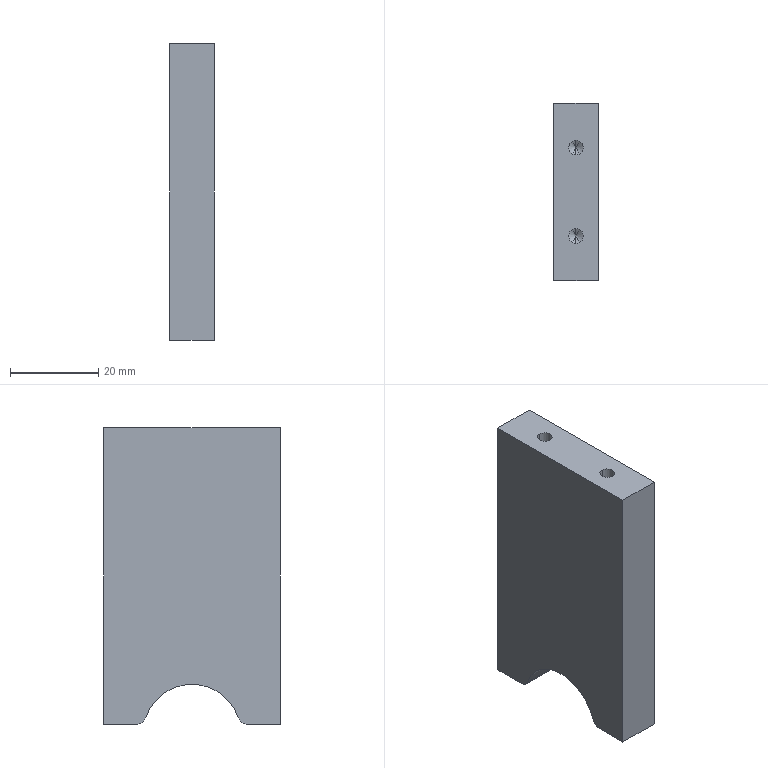Component | SolidWorks | 09-1111-1 | 1 solid | 26 faces | box 10 x 40 x 67 mm | volume 24903 mm3 | cylinder 11 | cone 8 | plane 7 | commonest cylinder face diameters 3.3 x8 4 x2 22 x1 | material AL6061(GB)Natural Anodized
build123d program:
from build123d import *

# Parameters (mm, degrees)
SKETCH1_W             = 67
SKETCH1_H             = 10
EXTRUDE1_DEPTH        = 40
SKETCH2_R             = 11
CUT_EXTRUDE1_DEPTH    = 79.67
M4_TAPPED_HOLE1_D     = 3.3
M4_TAPPED_HOLE1_DEPTH = 12.1
M4_TAPPED_HOLE1_TIP   = 0.9914
M4_TAPPED_HOLE2_D     = 3.3
M4_TAPPED_HOLE2_DEPTH = 12.1
M4_TAPPED_HOLE2_TIP   = 0.9914
FILLET1_R             = 2


with BuildPart() as part:
    # Sketch1 → Extrude1 (new body)
    with BuildSketch(Plane.XY):
        with Locations((33.5, 5)):
            Rectangle(SKETCH1_W, SKETCH1_H)
    extrude(amount=EXTRUDE1_DEPTH)

    # Sketch2 → Cut-Extrude1 (cut, through all)
    with BuildSketch(Plane(origin=(0, 10, 0), x_dir=(1, 0, 0), z_dir=(0, 1, 0))):
        with Locations((-2, -20)):
            Circle(SKETCH2_R)
    extrude(amount=-CUT_EXTRUDE1_DEPTH, mode=Mode.SUBTRACT)

    # M4 Tapped Hole1
    with Locations(Plane(origin=(67, 0, 0), x_dir=(0, 0, -1), z_dir=(1, 0, 0))):
        with Locations((-30, 5), (-10, 5)):
            Hole(M4_TAPPED_HOLE1_D / 2, depth=M4_TAPPED_HOLE1_DEPTH)
            with Locations((0, 0, -(M4_TAPPED_HOLE1_DEPTH + M4_TAPPED_HOLE1_TIP / 2))):  # 118° drill point
                Cone(0, M4_TAPPED_HOLE1_D / 2, M4_TAPPED_HOLE1_TIP, mode=Mode.SUBTRACT)

    # M4 Tapped Hole2
    with Locations(Plane(origin=(0, 5, 3.5), x_dir=(0, 0, -1), z_dir=(-1, 0, 0))):
        with Locations((0, 0), (-33, 0)):
            Hole(M4_TAPPED_HOLE2_D / 2, depth=M4_TAPPED_HOLE2_DEPTH)
            with Locations((0, 0, -(M4_TAPPED_HOLE2_DEPTH + M4_TAPPED_HOLE2_TIP / 2))):  # 118° drill point
                Cone(0, M4_TAPPED_HOLE2_D / 2, M4_TAPPED_HOLE2_TIP, mode=Mode.SUBTRACT)

    # Fillet1
    fillet1_edges = [part.edges().sort_by_distance(p)[0] for p in [
        (0, 5, 9.183),
        (0, 5, 30.817),
    ]]
    fillet(fillet1_edges, radius=FILLET1_R)


solid = part.part

# Placed as in the assembly
solid = solid.moved(Location((105, -35, -73), (90, 0, 90)))
STEP:
#1=CARTESIAN_POINT('',(3.937,-2.88,-2.398));
#2=VERTEX_POINT('',#1);
#3=CARTESIAN_POINT('',(3.937,-2.75,-2.398));
#4=VERTEX_POINT('',#3);
#5=CARTESIAN_POINT('',(3.937,-2.815,-2.398));
#6=DIRECTION('',(0.,-0.,-1.));
#7=DIRECTION('',(0.,1.,0.));
#8=AXIS2_PLACEMENT_3D('',#5,#6,#7);
#9=CIRCLE('',#8,0.06496);
#10=EDGE_CURVE('',#2,#4,#9,.T.);
#11=ORIENTED_EDGE('',*,*,#10,.F.);
#12=CARTESIAN_POINT('',(3.937,-2.88,-2.874));
#13=VERTEX_POINT('',#12);
#14=CARTESIAN_POINT('',(3.937,-2.88,-2.874));
#15=DIRECTION('',(0.,-0.,-1.));
#16=VECTOR('',#15,39.37);
#17=LINE('',#14,#16);
#18=EDGE_CURVE('',#2,#13,#17,.T.);
#19=ORIENTED_EDGE('',*,*,#18,.T.);
#20=CARTESIAN_POINT('',(3.937,-2.75,-2.874));
#21=VERTEX_POINT('',#20);
#22=CARTESIAN_POINT('',(3.937,-2.815,-2.874));
#23=DIRECTION('',(0.,-0.,-1.));
#24=DIRECTION('',(0.,1.,0.));
#25=AXIS2_PLACEMENT_3D('',#22,#23,#24);
#26=CIRCLE('',#25,0.06496);
#27=EDGE_CURVE('',#13,#21,#26,.T.);
#28=ORIENTED_EDGE('',*,*,#27,.T.);
#29=CARTESIAN_POINT('',(3.937,-2.75,-2.874));
#30=DIRECTION('',(0.,-0.,-1.));
#31=VECTOR('',#30,39.37);
#32=LINE('',#29,#31);
#33=EDGE_CURVE('',#4,#21,#32,.T.);
#34=ORIENTED_EDGE('',*,*,#33,.F.);
#35=EDGE_LOOP('',(#11,#19,#28,#34));
#36=FACE_OUTER_BOUND('',#35,.T.);
#37=CARTESIAN_POINT('',(3.937,-2.815,-2.874));
#38=DIRECTION('',(0.,-0.,-1.));
#39=DIRECTION('',(0.,1.,0.));
#40=AXIS2_PLACEMENT_3D('',#37,#38,#39);
#41=CYLINDRICAL_SURFACE('',#40,0.06496);
#42=ADVANCED_FACE('',(#36),#41,.F.);
#43=CARTESIAN_POINT('',(3.937,-2.815,-2.359));
#44=VERTEX_POINT('',#43);
#45=CARTESIAN_POINT('',(3.937,-2.75,-2.398));
#46=DIRECTION('',(0.,0.8572,-0.515));
#47=VECTOR('',#46,39.37);
#48=LINE('',#45,#47);
#49=EDGE_CURVE('',#44,#4,#48,.T.);
#50=ORIENTED_EDGE('',*,*,#49,.F.);
#51=CARTESIAN_POINT('',(3.937,-2.88,-2.398));
#52=DIRECTION('',(0.,-0.8572,-0.515));
#53=VECTOR('',#52,39.37);
#54=LINE('',#51,#53);
#55=EDGE_CURVE('',#44,#2,#54,.T.);
#56=ORIENTED_EDGE('',*,*,#55,.T.);
#57=ORIENTED_EDGE('',*,*,#10,.T.);
#58=EDGE_LOOP('',(#50,#56,#57));
#59=FACE_OUTER_BOUND('',#58,.T.);
#60=CARTESIAN_POINT('',(3.937,-2.815,-2.398));
#61=DIRECTION('',(0.,-0.,-1.));
#62=DIRECTION('',(0.,1.,0.));
#63=AXIS2_PLACEMENT_3D('',#60,#61,#62);
#64=CONICAL_SURFACE('',#63,0.06496,1.03);
#65=ADVANCED_FACE('',(#59),#64,.F.);
#66=CARTESIAN_POINT('',(3.937,-1.581,-2.398));
#67=VERTEX_POINT('',#66);
#68=CARTESIAN_POINT('',(3.937,-1.451,-2.398));
#69=VERTEX_POINT('',#68);
#70=CARTESIAN_POINT('',(3.937,-1.516,-2.398));
#71=DIRECTION('',(0.,-0.,-1.));
#72=DIRECTION('',(0.,1.,0.));
#73=AXIS2_PLACEMENT_3D('',#70,#71,#72);
#74=CIRCLE('',#73,0.06496);
#75=EDGE_CURVE('',#67,#69,#74,.T.);
#76=ORIENTED_EDGE('',*,*,#75,.F.);
#77=CARTESIAN_POINT('',(3.937,-1.581,-2.874));
#78=VERTEX_POINT('',#77);
#79=CARTESIAN_POINT('',(3.937,-1.581,-2.874));
#80=DIRECTION('',(0.,-0.,-1.));
#81=VECTOR('',#80,39.37);
#82=LINE('',#79,#81);
#83=EDGE_CURVE('',#67,#78,#82,.T.);
#84=ORIENTED_EDGE('',*,*,#83,.T.);
#85=CARTESIAN_POINT('',(3.937,-1.451,-2.874));
#86=VERTEX_POINT('',#85);
#87=CARTESIAN_POINT('',(3.937,-1.516,-2.874));
#88=DIRECTION('',(0.,-0.,-1.));
#89=DIRECTION('',(0.,1.,0.));
#90=AXIS2_PLACEMENT_3D('',#87,#88,#89);
#91=CIRCLE('',#90,0.06496);
#92=EDGE_CURVE('',#78,#86,#91,.T.);
#93=ORIENTED_EDGE('',*,*,#92,.T.);
#94=CARTESIAN_POINT('',(3.937,-1.451,-2.874));
#95=DIRECTION('',(0.,-0.,-1.));
#96=VECTOR('',#95,39.37);
#97=LINE('',#94,#96);
#98=EDGE_CURVE('',#69,#86,#97,.T.);
#99=ORIENTED_EDGE('',*,*,#98,.F.);
#100=EDGE_LOOP('',(#76,#84,#93,#99));
#101=FACE_OUTER_BOUND('',#100,.T.);
#102=CARTESIAN_POINT('',(3.937,-1.516,-2.874));
#103=DIRECTION('',(0.,-0.,-1.));
#104=DIRECTION('',(0.,1.,0.));
#105=AXIS2_PLACEMENT_3D('',#102,#103,#104);
#106=CYLINDRICAL_SURFACE('',#105,0.06496);
#107=ADVANCED_FACE('',(#101),#106,.F.);
#108=CARTESIAN_POINT('',(3.937,-1.516,-2.359));
#109=VERTEX_POINT('',#108);
#110=CARTESIAN_POINT('',(3.937,-1.451,-2.398));
#111=DIRECTION('',(0.,0.8572,-0.515));
#112=VECTOR('',#111,39.37);
#113=LINE('',#110,#112);
#114=EDGE_CURVE('',#109,#69,#113,.T.);
#115=ORIENTED_EDGE('',*,*,#114,.F.);
#116=CARTESIAN_POINT('',(3.937,-1.581,-2.398));
#117=DIRECTION('',(0.,-0.8572,-0.515));
#118=VECTOR('',#117,39.37);
#119=LINE('',#116,#118);
#120=EDGE_CURVE('',#109,#67,#119,.T.);
#121=ORIENTED_EDGE('',*,*,#120,.T.);
#122=ORIENTED_EDGE('',*,*,#75,.T.);
#123=EDGE_LOOP('',(#115,#121,#122));
#124=FACE_OUTER_BOUND('',#123,.T.);
#125=CARTESIAN_POINT('',(3.937,-1.516,-2.398));
#126=DIRECTION('',(0.,-0.,-1.));
#127=DIRECTION('',(0.,1.,0.));
#128=AXIS2_PLACEMENT_3D('',#125,#126,#127);
#129=CONICAL_SURFACE('',#128,0.06496,1.03);
#130=ADVANCED_FACE('',(#124),#129,.F.);
#131=CARTESIAN_POINT('',(3.937,-1.707,-0.7126));
#132=VERTEX_POINT('',#131);
#133=CARTESIAN_POINT('',(3.937,-1.837,-0.7126));
#134=VERTEX_POINT('',#133);
#135=CARTESIAN_POINT('',(3.937,-1.772,-0.7126));
#136=DIRECTION('',(-0.,0.,1.));
#137=DIRECTION('',(0.,-1.,0.));
#138=AXIS2_PLACEMENT_3D('',#135,#136,#137);
#139=CIRCLE('',#138,0.06496);
#140=EDGE_CURVE('',#132,#134,#139,.T.);
#141=ORIENTED_EDGE('',*,*,#140,.F.);
#142=CARTESIAN_POINT('',(3.937,-1.707,-0.2362));
#143=VERTEX_POINT('',#142);
#144=CARTESIAN_POINT('',(3.937,-1.707,-0.2362));
#145=DIRECTION('',(-0.,0.,1.));
#146=VECTOR('',#145,39.37);
#147=LINE('',#144,#146);
#148=EDGE_CURVE('',#132,#143,#147,.T.);
#149=ORIENTED_EDGE('',*,*,#148,.T.);
#150=CARTESIAN_POINT('',(3.937,-1.837,-0.2362));
#151=VERTEX_POINT('',#150);
#152=CARTESIAN_POINT('',(3.937,-1.772,-0.2362));
#153=DIRECTION('',(-0.,0.,1.));
#154=DIRECTION('',(0.,-1.,0.));
#155=AXIS2_PLACEMENT_3D('',#152,#153,#154);
#156=CIRCLE('',#155,0.06496);
#157=EDGE_CURVE('',#143,#151,#156,.T.);
#158=ORIENTED_EDGE('',*,*,#157,.T.);
#159=CARTESIAN_POINT('',(3.937,-1.837,-0.2362));
#160=DIRECTION('',(-0.,0.,1.));
#161=VECTOR('',#160,39.37);
#162=LINE('',#159,#161);
#163=EDGE_CURVE('',#134,#151,#162,.T.);
#164=ORIENTED_EDGE('',*,*,#163,.F.);
#165=EDGE_LOOP('',(#141,#149,#158,#164));
#166=FACE_OUTER_BOUND('',#165,.T.);
#167=CARTESIAN_POINT('',(3.937,-1.772,-0.2362));
#168=DIRECTION('',(-0.,0.,1.));
#169=DIRECTION('',(0.,-1.,0.));
#170=AXIS2_PLACEMENT_3D('',#167,#168,#169);
#171=CYLINDRICAL_SURFACE('',#170,0.06496);
#172=ADVANCED_FACE('',(#166),#171,.F.);
#173=CARTESIAN_POINT('',(3.937,-1.772,-0.7516));
#174=VERTEX_POINT('',#173);
#175=CARTESIAN_POINT('',(3.937,-1.837,-0.7126));
#176=DIRECTION('',(-0.,-0.8572,0.515));
#177=VECTOR('',#176,39.37);
#178=LINE('',#175,#177);
#179=EDGE_CURVE('',#174,#134,#178,.T.);
#180=ORIENTED_EDGE('',*,*,#179,.F.);
#181=CARTESIAN_POINT('',(3.937,-1.707,-0.7126));
#182=DIRECTION('',(0.,0.8572,0.515));
#183=VECTOR('',#182,39.37);
#184=LINE('',#181,#183);
#185=EDGE_CURVE('',#174,#132,#184,.T.);
#186=ORIENTED_EDGE('',*,*,#185,.T.);
#187=ORIENTED_EDGE('',*,*,#140,.T.);
#188=EDGE_LOOP('',(#180,#186,#187));
#189=FACE_OUTER_BOUND('',#188,.T.);
#190=CARTESIAN_POINT('',(3.937,-1.772,-0.7126));
#191=DIRECTION('',(-0.,0.,1.));
#192=DIRECTION('',(0.,-1.,0.));
#193=AXIS2_PLACEMENT_3D('',#190,#191,#192);
#194=CONICAL_SURFACE('',#193,0.06496,1.03);
#195=ADVANCED_FACE('',(#189),#194,.F.);
#196=CARTESIAN_POINT('',(3.937,-2.494,-0.7126));
#197=VERTEX_POINT('',#196);
#198=CARTESIAN_POINT('',(3.937,-2.624,-0.7126));
#199=VERTEX_POINT('',#198);
#200=CARTESIAN_POINT('',(3.937,-2.559,-0.7126));
#201=DIRECTION('',(-0.,0.,1.));
#202=DIRECTION('',(0.,-1.,0.));
#203=AXIS2_PLACEMENT_3D('',#200,#201,#202);
#204=CIRCLE('',#203,0.06496);
#205=EDGE_CURVE('',#197,#199,#204,.T.);
#206=ORIENTED_EDGE('',*,*,#205,.F.);
#207=CARTESIAN_POINT('',(3.937,-2.494,-0.2362));
#208=VERTEX_POINT('',#207);
#209=CARTESIAN_POINT('',(3.937,-2.494,-0.2362));
#210=DIRECTION('',(-0.,0.,1.));
#211=VECTOR('',#210,39.37);
#212=LINE('',#209,#211);
#213=EDGE_CURVE('',#197,#208,#212,.T.);
#214=ORIENTED_EDGE('',*,*,#213,.T.);
#215=CARTESIAN_POINT('',(3.937,-2.624,-0.2362));
#216=VERTEX_POINT('',#215);
#217=CARTESIAN_POINT('',(3.937,-2.559,-0.2362));
#218=DIRECTION('',(-0.,0.,1.));
#219=DIRECTION('',(0.,-1.,0.));
#220=AXIS2_PLACEMENT_3D('',#217,#218,#219);
#221=CIRCLE('',#220,0.06496);
#222=EDGE_CURVE('',#208,#216,#221,.T.);
#223=ORIENTED_EDGE('',*,*,#222,.T.);
#224=CARTESIAN_POINT('',(3.937,-2.624,-0.2362));
#225=DIRECTION('',(-0.,0.,1.));
#226=VECTOR('',#225,39.37);
#227=LINE('',#224,#226);
#228=EDGE_CURVE('',#199,#216,#227,.T.);
#229=ORIENTED_EDGE('',*,*,#228,.F.);
#230=EDGE_LOOP('',(#206,#214,#223,#229));
#231=FACE_OUTER_BOUND('',#230,.T.);
#232=CARTESIAN_POINT('',(3.937,-2.559,-0.2362));
#233=DIRECTION('',(-0.,0.,1.));
#234=DIRECTION('',(0.,-1.,0.));
#235=AXIS2_PLACEMENT_3D('',#232,#233,#234);
#236=CYLINDRICAL_SURFACE('',#235,0.06496);
#237=ADVANCED_FACE('',(#231),#236,.F.);
#238=CARTESIAN_POINT('',(3.937,-2.559,-0.7516));
#239=VERTEX_POINT('',#238);
#240=CARTESIAN_POINT('',(3.937,-2.624,-0.7126));
#241=DIRECTION('',(-0.,-0.8572,0.515));
#242=VECTOR('',#241,39.37);
#243=LINE('',#240,#242);
#244=EDGE_CURVE('',#239,#199,#243,.T.);
#245=ORIENTED_EDGE('',*,*,#244,.F.);
#246=CARTESIAN_POINT('',(3.937,-2.494,-0.7126));
#247=DIRECTION('',(0.,0.8572,0.515));
#248=VECTOR('',#247,39.37);
#249=LINE('',#246,#248);
#250=EDGE_CURVE('',#239,#197,#249,.T.);
#251=ORIENTED_EDGE('',*,*,#250,.T.);
#252=ORIENTED_EDGE('',*,*,#205,.T.);
#253=EDGE_LOOP('',(#245,#251,#252));
#254=FACE_OUTER_BOUND('',#253,.T.);
#255=CARTESIAN_POINT('',(3.937,-2.559,-0.7126));
#256=DIRECTION('',(-0.,0.,1.));
#257=DIRECTION('',(0.,-1.,0.));
#258=AXIS2_PLACEMENT_3D('',#255,#256,#257);
#259=CONICAL_SURFACE('',#258,0.06496,1.03);
#260=ADVANCED_FACE('',(#254),#259,.F.);
#261=CARTESIAN_POINT('',(3.937,-2.815,-2.874));
#262=DIRECTION('',(0.,-0.,-1.));
#263=DIRECTION('',(0.,1.,0.));
#264=AXIS2_PLACEMENT_3D('',#261,#262,#263);
#265=CIRCLE('',#264,0.06496);
#266=EDGE_CURVE('',#21,#13,#265,.T.);
#267=ORIENTED_EDGE('',*,*,#266,.F.);
#268=ORIENTED_EDGE('',*,*,#27,.F.);
#269=EDGE_LOOP('',(#267,#268));
#270=FACE_BOUND('',#269,.T.);
#271=CARTESIAN_POINT('',(3.74,-2.652,-2.874));
#272=VERTEX_POINT('',#271);
#273=CARTESIAN_POINT('',(3.74,-2.953,-2.874));
#274=VERTEX_POINT('',#273);
#275=CARTESIAN_POINT('',(3.74,-1.378,-2.874));
#276=DIRECTION('',(-0.,-1.,0.));
#277=VECTOR('',#276,39.37);
#278=LINE('',#275,#277);
#279=EDGE_CURVE('',#272,#274,#278,.T.);
#280=ORIENTED_EDGE('',*,*,#279,.F.);
#281=CARTESIAN_POINT('',(4.134,-2.652,-2.874));
#282=VERTEX_POINT('',#281);
#283=CARTESIAN_POINT('',(3.74,-2.652,-2.874));
#284=DIRECTION('',(1.,-0.,0.));
#285=VECTOR('',#284,39.37);
#286=LINE('',#283,#285);
#287=EDGE_CURVE('',#272,#282,#286,.T.);
#288=ORIENTED_EDGE('',*,*,#287,.T.);
#289=CARTESIAN_POINT('',(4.134,-2.953,-2.874));
#290=VERTEX_POINT('',#289);
#291=CARTESIAN_POINT('',(4.134,-1.378,-2.874));
#292=DIRECTION('',(-0.,-1.,0.));
#293=VECTOR('',#292,39.37);
#294=LINE('',#291,#293);
#295=EDGE_CURVE('',#282,#290,#294,.T.);
#296=ORIENTED_EDGE('',*,*,#295,.T.);
#297=CARTESIAN_POINT('',(3.74,-2.953,-2.874));
#298=DIRECTION('',(-1.,0.,-0.));
#299=VECTOR('',#298,39.37);
#300=LINE('',#297,#299);
#301=EDGE_CURVE('',#290,#274,#300,.T.);
#302=ORIENTED_EDGE('',*,*,#301,.T.);
#303=EDGE_LOOP('',(#280,#288,#296,#302));
#304=FACE_OUTER_BOUND('',#303,.T.);
#305=CARTESIAN_POINT('',(3.74,-1.378,-2.874));
#306=DIRECTION('',(-0.,0.,1.));
#307=DIRECTION('',(-0.,-1.,0.));
#308=AXIS2_PLACEMENT_3D('',#305,#306,#307);
#309=PLANE('',#308);
#310=ADVANCED_FACE('',(#270,#304),#309,.F.);
#311=CARTESIAN_POINT('',(3.937,-1.516,-2.874));
#312=DIRECTION('',(0.,-0.,-1.));
#313=DIRECTION('',(0.,1.,0.));
#314=AXIS2_PLACEMENT_3D('',#311,#312,#313);
#315=CIRCLE('',#314,0.06496);
#316=EDGE_CURVE('',#86,#78,#315,.T.);
#317=ORIENTED_EDGE('',*,*,#316,.F.);
#318=ORIENTED_EDGE('',*,*,#92,.F.);
#319=EDGE_LOOP('',(#317,#318));
#320=FACE_BOUND('',#319,.T.);
#321=CARTESIAN_POINT('',(4.134,-1.378,-2.874));
#322=VERTEX_POINT('',#321);
#323=CARTESIAN_POINT('',(4.134,-1.678,-2.874));
#324=VERTEX_POINT('',#323);
#325=CARTESIAN_POINT('',(4.134,-1.378,-2.874));
#326=DIRECTION('',(-0.,-1.,0.));
#327=VECTOR('',#326,39.37);
#328=LINE('',#325,#327);
#329=EDGE_CURVE('',#322,#324,#328,.T.);
#330=ORIENTED_EDGE('',*,*,#329,.T.);
#331=CARTESIAN_POINT('',(3.74,-1.678,-2.874));
#332=VERTEX_POINT('',#331);
#333=CARTESIAN_POINT('',(3.74,-1.678,-2.874));
#334=DIRECTION('',(-1.,0.,-0.));
#335=VECTOR('',#334,39.37);
#336=LINE('',#333,#335);
#337=EDGE_CURVE('',#324,#332,#336,.T.);
#338=ORIENTED_EDGE('',*,*,#337,.T.);
#339=CARTESIAN_POINT('',(3.74,-1.378,-2.874));
#340=VERTEX_POINT('',#339);
#341=CARTESIAN_POINT('',(3.74,-1.378,-2.874));
#342=DIRECTION('',(-0.,-1.,0.));
#343=VECTOR('',#342,39.37);
#344=LINE('',#341,#343);
#345=EDGE_CURVE('',#340,#332,#344,.T.);
#346=ORIENTED_EDGE('',*,*,#345,.F.);
#347=CARTESIAN_POINT('',(3.74,-1.378,-2.874));
#348=DIRECTION('',(-1.,0.,-0.));
#349=VECTOR('',#348,39.37);
#350=LINE('',#347,#349);
#351=EDGE_CURVE('',#322,#340,#350,.T.);
#352=ORIENTED_EDGE('',*,*,#351,.F.);
#353=EDGE_LOOP('',(#330,#338,#346,#352));
#354=FACE_OUTER_BOUND('',#353,.T.);
#355=CARTESIAN_POINT('',(3.74,-1.378,-2.874));
#356=DIRECTION('',(-0.,0.,1.));
#357=DIRECTION('',(-0.,-1.,0.));
#358=AXIS2_PLACEMENT_3D('',#355,#356,#357);
#359=PLANE('',#358);
#360=ADVANCED_FACE('',(#320,#354),#359,.F.);
#361=ORIENTED_EDGE('',*,*,#345,.T.);
#362=CARTESIAN_POINT('',(3.74,-1.753,-2.82));
#363=VERTEX_POINT('',#362);
#364=CARTESIAN_POINT('',(3.74,-1.678,-2.795));
#365=DIRECTION('',(-1.,0.,-0.));
#366=DIRECTION('',(0.,1.,0.));
#367=AXIS2_PLACEMENT_3D('',#364,#365,#366);
#368=CIRCLE('',#367,0.07874);
#369=EDGE_CURVE('',#332,#363,#368,.T.);
#370=ORIENTED_EDGE('',*,*,#369,.T.);
#371=CARTESIAN_POINT('',(3.74,-2.577,-2.82));
#372=VERTEX_POINT('',#371);
#373=CARTESIAN_POINT('',(3.74,-2.165,-2.953));
#374=DIRECTION('',(1.,-0.,0.));
#375=DIRECTION('',(0.,1.,0.));
#376=AXIS2_PLACEMENT_3D('',#373,#374,#375);
#377=CIRCLE('',#376,0.4331);
#378=EDGE_CURVE('',#363,#372,#377,.T.);
#379=ORIENTED_EDGE('',*,*,#378,.T.);
#380=CARTESIAN_POINT('',(3.74,-2.652,-2.795));
#381=DIRECTION('',(-1.,0.,-0.));
#382=DIRECTION('',(0.,1.,0.));
#383=AXIS2_PLACEMENT_3D('',#380,#381,#382);
#384=CIRCLE('',#383,0.07874);
#385=EDGE_CURVE('',#372,#272,#384,.T.);
#386=ORIENTED_EDGE('',*,*,#385,.T.);
#387=ORIENTED_EDGE('',*,*,#279,.T.);
#388=CARTESIAN_POINT('',(3.74,-2.953,-0.2362));
#389=VERTEX_POINT('',#388);
#390=CARTESIAN_POINT('',(3.74,-2.953,-2.874));
#391=DIRECTION('',(-0.,0.,1.));
#392=VECTOR('',#391,39.37);
#393=LINE('',#390,#392);
#394=EDGE_CURVE('',#274,#389,#393,.T.);
#395=ORIENTED_EDGE('',*,*,#394,.T.);
#396=CARTESIAN_POINT('',(3.74,-1.378,-0.2362));
#397=VERTEX_POINT('',#396);
#398=CARTESIAN_POINT('',(3.74,-1.378,-0.2362));
#399=DIRECTION('',(-0.,-1.,0.));
#400=VECTOR('',#399,39.37);
#401=LINE('',#398,#400);
#402=EDGE_CURVE('',#397,#389,#401,.T.);
#403=ORIENTED_EDGE('',*,*,#402,.F.);
#404=CARTESIAN_POINT('',(3.74,-1.378,-2.874));
#405=DIRECTION('',(-0.,0.,1.));
#406=VECTOR('',#405,39.37);
#407=LINE('',#404,#406);
#408=EDGE_CURVE('',#340,#397,#407,.T.);
#409=ORIENTED_EDGE('',*,*,#408,.F.);
#410=EDGE_LOOP('',(#361,#370,#379,#386,#387,#395,#403,#409));
#411=FACE_OUTER_BOUND('',#410,.T.);
#412=CARTESIAN_POINT('',(3.74,-1.378,-2.874));
#413=DIRECTION('',(1.,-0.,0.));
#414=DIRECTION('',(0.,1.,-0.));
#415=AXIS2_PLACEMENT_3D('',#412,#413,#414);
#416=PLANE('',#415);
#417=ADVANCED_FACE('',(#411),#416,.F.);
#418=CARTESIAN_POINT('',(3.937,-1.772,-0.2362));
#419=DIRECTION('',(-0.,0.,1.));
#420=DIRECTION('',(0.,-1.,0.));
#421=AXIS2_PLACEMENT_3D('',#418,#419,#420);
#422=CIRCLE('',#421,0.06496);
#423=EDGE_CURVE('',#151,#143,#422,.T.);
#424=ORIENTED_EDGE('',*,*,#423,.F.);
#425=ORIENTED_EDGE('',*,*,#157,.F.);
#426=EDGE_LOOP('',(#424,#425));
#427=FACE_BOUND('',#426,.T.);
#428=CARTESIAN_POINT('',(3.937,-2.559,-0.2362));
#429=DIRECTION('',(-0.,0.,1.));
#430=DIRECTION('',(0.,-1.,0.));
#431=AXIS2_PLACEMENT_3D('',#428,#429,#430);
#432=CIRCLE('',#431,0.06496);
#433=EDGE_CURVE('',#216,#208,#432,.T.);
#434=ORIENTED_EDGE('',*,*,#433,.F.);
#435=ORIENTED_EDGE('',*,*,#222,.F.);
#436=EDGE_LOOP('',(#434,#435));
#437=FACE_BOUND('',#436,.T.);
#438=CARTESIAN_POINT('',(4.134,-2.953,-0.2362));
#439=VERTEX_POINT('',#438);
#440=CARTESIAN_POINT('',(3.74,-2.953,-0.2362));
#441=DIRECTION('',(1.,-0.,0.));
#442=VECTOR('',#441,39.37);
#443=LINE('',#440,#442);
#444=EDGE_CURVE('',#389,#439,#443,.T.);
#445=ORIENTED_EDGE('',*,*,#444,.T.);
#446=CARTESIAN_POINT('',(4.134,-1.378,-0.2362));
#447=VERTEX_POINT('',#446);
#448=CARTESIAN_POINT('',(4.134,-1.378,-0.2362));
#449=DIRECTION('',(-0.,-1.,0.));
#450=VECTOR('',#449,39.37);
#451=LINE('',#448,#450);
#452=EDGE_CURVE('',#447,#439,#451,.T.);
#453=ORIENTED_EDGE('',*,*,#452,.F.);
#454=CARTESIAN_POINT('',(3.74,-1.378,-0.2362));
#455=DIRECTION('',(1.,-0.,0.));
#456=VECTOR('',#455,39.37);
#457=LINE('',#454,#456);
#458=EDGE_CURVE('',#397,#447,#457,.T.);
#459=ORIENTED_EDGE('',*,*,#458,.F.);
#460=ORIENTED_EDGE('',*,*,#402,.T.);
#461=EDGE_LOOP('',(#445,#453,#459,#460));
#462=FACE_OUTER_BOUND('',#461,.T.);
#463=CARTESIAN_POINT('',(3.74,-1.378,-0.2362));
#464=DIRECTION('',(0.,-0.,-1.));
#465=DIRECTION('',(0.,1.,-0.));
#466=AXIS2_PLACEMENT_3D('',#463,#464,#465);
#467=PLANE('',#466);
#468=ADVANCED_FACE('',(#427,#437,#462),#467,.F.);
#469=CARTESIAN_POINT('',(4.134,-1.753,-2.82));
#470=VERTEX_POINT('',#469);
#471=CARTESIAN_POINT('',(4.134,-2.577,-2.82));
#472=VERTEX_POINT('',#471);
#473=CARTESIAN_POINT('',(4.134,-2.165,-2.953));
#474=DIRECTION('',(1.,-0.,0.));
#475=DIRECTION('',(0.,1.,0.));
#476=AXIS2_PLACEMENT_3D('',#473,#474,#475);
#477=CIRCLE('',#476,0.4331);
#478=EDGE_CURVE('',#470,#472,#477,.T.);
#479=ORIENTED_EDGE('',*,*,#478,.F.);
#480=CARTESIAN_POINT('',(4.134,-1.678,-2.795));
#481=DIRECTION('',(1.,-0.,0.));
#482=DIRECTION('',(0.,-1.,0.));
#483=AXIS2_PLACEMENT_3D('',#480,#481,#482);
#484=CIRCLE('',#483,0.07874);
#485=EDGE_CURVE('',#470,#324,#484,.T.);
#486=ORIENTED_EDGE('',*,*,#485,.T.);
#487=ORIENTED_EDGE('',*,*,#329,.F.);
#488=CARTESIAN_POINT('',(4.134,-1.378,-2.874));
#489=DIRECTION('',(0.,-0.,-1.));
#490=VECTOR('',#489,39.37);
#491=LINE('',#488,#490);
#492=EDGE_CURVE('',#447,#322,#491,.T.);
#493=ORIENTED_EDGE('',*,*,#492,.F.);
#494=ORIENTED_EDGE('',*,*,#452,.T.);
#495=CARTESIAN_POINT('',(4.134,-2.953,-2.874));
#496=DIRECTION('',(0.,-0.,-1.));
#497=VECTOR('',#496,39.37);
#498=LINE('',#495,#497);
#499=EDGE_CURVE('',#439,#290,#498,.T.);
#500=ORIENTED_EDGE('',*,*,#499,.T.);
#501=ORIENTED_EDGE('',*,*,#295,.F.);
#502=CARTESIAN_POINT('',(4.134,-2.652,-2.795));
#503=DIRECTION('',(1.,-0.,0.));
#504=DIRECTION('',(0.,-1.,0.));
#505=AXIS2_PLACEMENT_3D('',#502,#503,#504);
#506=CIRCLE('',#505,0.07874);
#507=EDGE_CURVE('',#282,#472,#506,.T.);
#508=ORIENTED_EDGE('',*,*,#507,.T.);
#509=EDGE_LOOP('',(#479,#486,#487,#493,#494,#500,#501,#508));
#510=FACE_OUTER_BOUND('',#509,.T.);
#511=CARTESIAN_POINT('',(4.134,-1.378,-2.874));
#512=DIRECTION('',(-1.,0.,-0.));
#513=DIRECTION('',(-0.,-1.,0.));
#514=AXIS2_PLACEMENT_3D('',#511,#512,#513);
#515=PLANE('',#514);
#516=ADVANCED_FACE('',(#510),#515,.F.);
#517=ORIENTED_EDGE('',*,*,#351,.T.);
#518=ORIENTED_EDGE('',*,*,#408,.T.);
#519=ORIENTED_EDGE('',*,*,#458,.T.);
#520=ORIENTED_EDGE('',*,*,#492,.T.);
#521=EDGE_LOOP('',(#517,#518,#519,#520));
#522=FACE_OUTER_BOUND('',#521,.T.);
#523=CARTESIAN_POINT('',(4.134,-1.378,-2.874));
#524=DIRECTION('',(-0.,-1.,0.));
#525=DIRECTION('',(0.,-0.,-1.));
#526=AXIS2_PLACEMENT_3D('',#523,#524,#525);
#527=PLANE('',#526);
#528=ADVANCED_FACE('',(#522),#527,.F.);
#529=ORIENTED_EDGE('',*,*,#301,.F.);
#530=ORIENTED_EDGE('',*,*,#499,.F.);
#531=ORIENTED_EDGE('',*,*,#444,.F.);
#532=ORIENTED_EDGE('',*,*,#394,.F.);
#533=EDGE_LOOP('',(#529,#530,#531,#532));
#534=FACE_OUTER_BOUND('',#533,.T.);
#535=CARTESIAN_POINT('',(4.134,-2.953,-2.874));
#536=DIRECTION('',(-0.,-1.,0.));
#537=DIRECTION('',(0.,-0.,-1.));
#538=AXIS2_PLACEMENT_3D('',#535,#536,#537);
#539=PLANE('',#538);
#540=ADVANCED_FACE('',(#534),#539,.T.);
#541=ORIENTED_EDGE('',*,*,#378,.F.);
#542=CARTESIAN_POINT('',(3.74,-1.753,-2.82));
#543=DIRECTION('',(1.,-0.,0.));
#544=VECTOR('',#543,39.37);
#545=LINE('',#542,#544);
#546=EDGE_CURVE('',#363,#470,#545,.T.);
#547=ORIENTED_EDGE('',*,*,#546,.T.);
#548=ORIENTED_EDGE('',*,*,#478,.T.);
#549=CARTESIAN_POINT('',(3.74,-2.577,-2.82));
#550=DIRECTION('',(-1.,0.,-0.));
#551=VECTOR('',#550,39.37);
#552=LINE('',#549,#551);
#553=EDGE_CURVE('',#472,#372,#552,.T.);
#554=ORIENTED_EDGE('',*,*,#553,.T.);
#555=EDGE_LOOP('',(#541,#547,#548,#554));
#556=FACE_OUTER_BOUND('',#555,.T.);
#557=CARTESIAN_POINT('',(3.74,-2.165,-2.953));
#558=DIRECTION('',(1.,-0.,0.));
#559=DIRECTION('',(0.,1.,0.));
#560=AXIS2_PLACEMENT_3D('',#557,#558,#559);
#561=CYLINDRICAL_SURFACE('',#560,0.4331);
#562=ADVANCED_FACE('',(#556),#561,.F.);
#563=ORIENTED_EDGE('',*,*,#250,.F.);
#564=ORIENTED_EDGE('',*,*,#244,.T.);
#565=CARTESIAN_POINT('',(3.937,-2.559,-0.7126));
#566=DIRECTION('',(-0.,0.,1.));
#567=DIRECTION('',(0.,-1.,0.));
#568=AXIS2_PLACEMENT_3D('',#565,#566,#567);
#569=CIRCLE('',#568,0.06496);
#570=EDGE_CURVE('',#199,#197,#569,.T.);
#571=ORIENTED_EDGE('',*,*,#570,.T.);
#572=EDGE_LOOP('',(#563,#564,#571));
#573=FACE_OUTER_BOUND('',#572,.T.);
#574=CARTESIAN_POINT('',(3.937,-2.559,-0.7126));
#575=DIRECTION('',(-0.,0.,1.));
#576=DIRECTION('',(0.,-1.,0.));
#577=AXIS2_PLACEMENT_3D('',#574,#575,#576);
#578=CONICAL_SURFACE('',#577,0.06496,1.03);
#579=ADVANCED_FACE('',(#573),#578,.F.);
#580=ORIENTED_EDGE('',*,*,#213,.F.);
#581=ORIENTED_EDGE('',*,*,#570,.F.);
#582=ORIENTED_EDGE('',*,*,#228,.T.);
#583=ORIENTED_EDGE('',*,*,#433,.T.);
#584=EDGE_LOOP('',(#580,#581,#582,#583));
#585=FACE_OUTER_BOUND('',#584,.T.);
#586=CARTESIAN_POINT('',(3.937,-2.559,-0.2362));
#587=DIRECTION('',(-0.,0.,1.));
#588=DIRECTION('',(0.,-1.,0.));
#589=AXIS2_PLACEMENT_3D('',#586,#587,#588);
#590=CYLINDRICAL_SURFACE('',#589,0.06496);
#591=ADVANCED_FACE('',(#585),#590,.F.);
#592=ORIENTED_EDGE('',*,*,#185,.F.);
#593=ORIENTED_EDGE('',*,*,#179,.T.);
#594=CARTESIAN_POINT('',(3.937,-1.772,-0.7126));
#595=DIRECTION('',(-0.,0.,1.));
#596=DIRECTION('',(0.,-1.,0.));
#597=AXIS2_PLACEMENT_3D('',#594,#595,#596);
#598=CIRCLE('',#597,0.06496);
#599=EDGE_CURVE('',#134,#132,#598,.T.);
#600=ORIENTED_EDGE('',*,*,#599,.T.);
#601=EDGE_LOOP('',(#592,#593,#600));
#602=FACE_OUTER_BOUND('',#601,.T.);
#603=CARTESIAN_POINT('',(3.937,-1.772,-0.7126));
#604=DIRECTION('',(-0.,0.,1.));
#605=DIRECTION('',(0.,-1.,0.));
#606=AXIS2_PLACEMENT_3D('',#603,#604,#605);
#607=CONICAL_SURFACE('',#606,0.06496,1.03);
#608=ADVANCED_FACE('',(#602),#607,.F.);
#609=ORIENTED_EDGE('',*,*,#148,.F.);
#610=ORIENTED_EDGE('',*,*,#599,.F.);
#611=ORIENTED_EDGE('',*,*,#163,.T.);
#612=ORIENTED_EDGE('',*,*,#423,.T.);
#613=EDGE_LOOP('',(#609,#610,#611,#612));
#614=FACE_OUTER_BOUND('',#613,.T.);
#615=CARTESIAN_POINT('',(3.937,-1.772,-0.2362));
#616=DIRECTION('',(-0.,0.,1.));
#617=DIRECTION('',(0.,-1.,0.));
#618=AXIS2_PLACEMENT_3D('',#615,#616,#617);
#619=CYLINDRICAL_SURFACE('',#618,0.06496);
#620=ADVANCED_FACE('',(#614),#619,.F.);
#621=ORIENTED_EDGE('',*,*,#120,.F.);
#622=ORIENTED_EDGE('',*,*,#114,.T.);
#623=CARTESIAN_POINT('',(3.937,-1.516,-2.398));
#624=DIRECTION('',(0.,-0.,-1.));
#625=DIRECTION('',(0.,1.,0.));
#626=AXIS2_PLACEMENT_3D('',#623,#624,#625);
#627=CIRCLE('',#626,0.06496);
#628=EDGE_CURVE('',#69,#67,#627,.T.);
#629=ORIENTED_EDGE('',*,*,#628,.T.);
#630=EDGE_LOOP('',(#621,#622,#629));
#631=FACE_OUTER_BOUND('',#630,.T.);
#632=CARTESIAN_POINT('',(3.937,-1.516,-2.398));
#633=DIRECTION('',(0.,-0.,-1.));
#634=DIRECTION('',(0.,1.,0.));
#635=AXIS2_PLACEMENT_3D('',#632,#633,#634);
#636=CONICAL_SURFACE('',#635,0.06496,1.03);
#637=ADVANCED_FACE('',(#631),#636,.F.);
#638=ORIENTED_EDGE('',*,*,#83,.F.);
#639=ORIENTED_EDGE('',*,*,#628,.F.);
#640=ORIENTED_EDGE('',*,*,#98,.T.);
#641=ORIENTED_EDGE('',*,*,#316,.T.);
#642=EDGE_LOOP('',(#638,#639,#640,#641));
#643=FACE_OUTER_BOUND('',#642,.T.);
#644=CARTESIAN_POINT('',(3.937,-1.516,-2.874));
#645=DIRECTION('',(0.,-0.,-1.));
#646=DIRECTION('',(0.,1.,0.));
#647=AXIS2_PLACEMENT_3D('',#644,#645,#646);
#648=CYLINDRICAL_SURFACE('',#647,0.06496);
#649=ADVANCED_FACE('',(#643),#648,.F.);
#650=ORIENTED_EDGE('',*,*,#55,.F.);
#651=ORIENTED_EDGE('',*,*,#49,.T.);
#652=CARTESIAN_POINT('',(3.937,-2.815,-2.398));
#653=DIRECTION('',(0.,-0.,-1.));
#654=DIRECTION('',(0.,1.,0.));
#655=AXIS2_PLACEMENT_3D('',#652,#653,#654);
#656=CIRCLE('',#655,0.06496);
#657=EDGE_CURVE('',#4,#2,#656,.T.);
#658=ORIENTED_EDGE('',*,*,#657,.T.);
#659=EDGE_LOOP('',(#650,#651,#658));
#660=FACE_OUTER_BOUND('',#659,.T.);
#661=CARTESIAN_POINT('',(3.937,-2.815,-2.398));
#662=DIRECTION('',(0.,-0.,-1.));
#663=DIRECTION('',(0.,1.,0.));
#664=AXIS2_PLACEMENT_3D('',#661,#662,#663);
#665=CONICAL_SURFACE('',#664,0.06496,1.03);
#666=ADVANCED_FACE('',(#660),#665,.F.);
#667=ORIENTED_EDGE('',*,*,#18,.F.);
#668=ORIENTED_EDGE('',*,*,#657,.F.);
#669=ORIENTED_EDGE('',*,*,#33,.T.);
#670=ORIENTED_EDGE('',*,*,#266,.T.);
#671=EDGE_LOOP('',(#667,#668,#669,#670));
#672=FACE_OUTER_BOUND('',#671,.T.);
#673=CARTESIAN_POINT('',(3.937,-2.815,-2.874));
#674=DIRECTION('',(0.,-0.,-1.));
#675=DIRECTION('',(0.,1.,0.));
#676=AXIS2_PLACEMENT_3D('',#673,#674,#675);
#677=CYLINDRICAL_SURFACE('',#676,0.06496);
#678=ADVANCED_FACE('',(#672),#677,.F.);
#679=ORIENTED_EDGE('',*,*,#485,.F.);
#680=ORIENTED_EDGE('',*,*,#546,.F.);
#681=ORIENTED_EDGE('',*,*,#369,.F.);
#682=ORIENTED_EDGE('',*,*,#337,.F.);
#683=EDGE_LOOP('',(#679,#680,#681,#682));
#684=FACE_OUTER_BOUND('',#683,.T.);
#685=CARTESIAN_POINT('',(3.74,-1.678,-2.795));
#686=DIRECTION('',(1.,-0.,0.));
#687=DIRECTION('',(0.,1.,0.));
#688=AXIS2_PLACEMENT_3D('',#685,#686,#687);
#689=CYLINDRICAL_SURFACE('',#688,0.07874);
#690=ADVANCED_FACE('',(#684),#689,.T.);
#691=ORIENTED_EDGE('',*,*,#385,.F.);
#692=ORIENTED_EDGE('',*,*,#553,.F.);
#693=ORIENTED_EDGE('',*,*,#507,.F.);
#694=ORIENTED_EDGE('',*,*,#287,.F.);
#695=EDGE_LOOP('',(#691,#692,#693,#694));
#696=FACE_OUTER_BOUND('',#695,.T.);
#697=CARTESIAN_POINT('',(3.74,-2.652,-2.795));
#698=DIRECTION('',(1.,-0.,0.));
#699=DIRECTION('',(0.,1.,0.));
#700=AXIS2_PLACEMENT_3D('',#697,#698,#699);
#701=CYLINDRICAL_SURFACE('',#700,0.07874);
#702=ADVANCED_FACE('',(#696),#701,.T.);
#703=CLOSED_SHELL('',(#42,#65,#107,#130,#172,#195,#237,#260,#310,#360,#417,#468,#516,#528,#540,#562,#579,#591,#608,#620,#637,#649,#666,#678,#690,#702));
#704=MANIFOLD_SOLID_BREP('',#703);
#705=CARTESIAN_POINT('',(0.,0.,0.));
#706=DIRECTION('',(0.,0.,1.));
#707=DIRECTION('',(1.,0.,0.));
#708=AXIS2_PLACEMENT_3D('',#705,#706,#707);
#709=(LENGTH_UNIT()NAMED_UNIT(*)SI_UNIT($,.METRE.));
#710=LENGTH_MEASURE_WITH_UNIT(LENGTH_MEASURE(0.0254),#709);
#711=DIMENSIONAL_EXPONENTS(1.,0.,0.,0.,0.,0.,0.);
#712=(CONVERSION_BASED_UNIT('',#710)LENGTH_UNIT()NAMED_UNIT(#711));
#713=UNCERTAINTY_MEASURE_WITH_UNIT(LENGTH_MEASURE(0.00001),#712,'','');
#714=(NAMED_UNIT(*)PLANE_ANGLE_UNIT()SI_UNIT($,.RADIAN.));
#715=(NAMED_UNIT(*)SI_UNIT($,.STERADIAN.)SOLID_ANGLE_UNIT());
#716=(GEOMETRIC_REPRESENTATION_CONTEXT(3)GLOBAL_UNCERTAINTY_ASSIGNED_CONTEXT((#713))GLOBAL_UNIT_ASSIGNED_CONTEXT((#712,#714,#715))REPRESENTATION_CONTEXT('',''));
#717=ADVANCED_BREP_SHAPE_REPRESENTATION('',(#704,#708),#716);
#718=COLOUR_RGB('',0.7922,0.8196,0.9333);
#719=FILL_AREA_STYLE_COLOUR('',#718);
#720=FILL_AREA_STYLE('',(#719));
#721=SURFACE_STYLE_FILL_AREA(#720);
#722=SURFACE_SIDE_STYLE('',(#721));
#723=SURFACE_STYLE_USAGE(.BOTH.,#722);
#724=PRESENTATION_STYLE_ASSIGNMENT((#723));
#725=STYLED_ITEM('',(#724),#704);
#726=PRESENTATION_LAYER_ASSIGNMENT('','',(#725));
#727=(LENGTH_UNIT()NAMED_UNIT(*)SI_UNIT($,.METRE.));
#728=LENGTH_MEASURE_WITH_UNIT(LENGTH_MEASURE(0.0254),#727);
#729=DIMENSIONAL_EXPONENTS(1.,0.,0.,0.,0.,0.,0.);
#730=(CONVERSION_BASED_UNIT('',#728)LENGTH_UNIT()NAMED_UNIT(#729));
#731=UNCERTAINTY_MEASURE_WITH_UNIT(LENGTH_MEASURE(0.00001),#730,'','');
#732=(NAMED_UNIT(*)PLANE_ANGLE_UNIT()SI_UNIT($,.RADIAN.));
#733=(NAMED_UNIT(*)SI_UNIT($,.STERADIAN.)SOLID_ANGLE_UNIT());
#734=(GEOMETRIC_REPRESENTATION_CONTEXT(3)GLOBAL_UNCERTAINTY_ASSIGNED_CONTEXT((#731))GLOBAL_UNIT_ASSIGNED_CONTEXT((#730,#732,#733))REPRESENTATION_CONTEXT('',''));
#735=MECHANICAL_DESIGN_GEOMETRIC_PRESENTATION_REPRESENTATION('',(#725),#734);